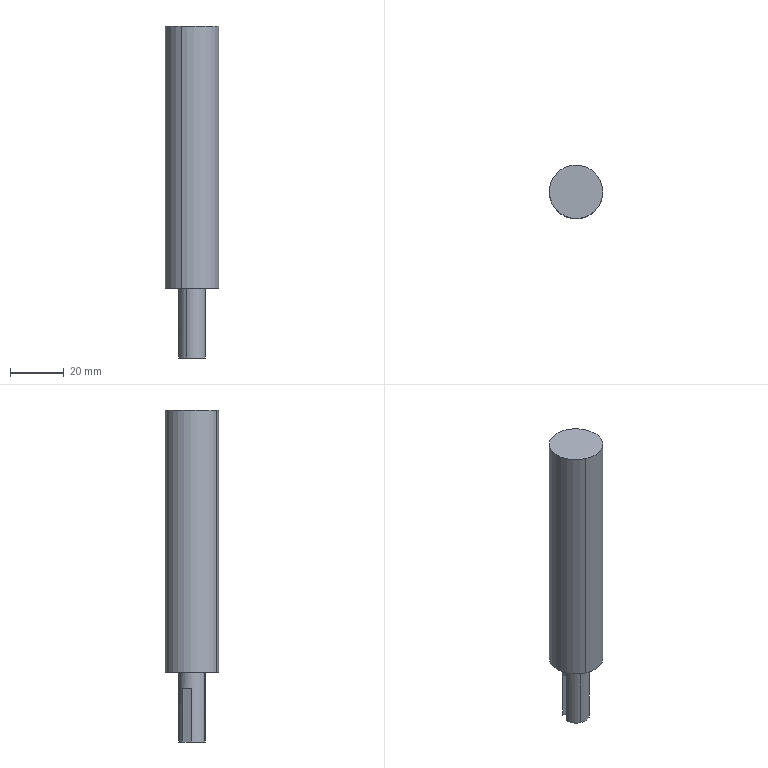Component | SolidWorks | DriveShaft-1 | 1 solid | 11 faces | box 20 x 20 x 124 mm | volume 32681 mm3 | plane 7 | cylinder 4 | commonest cylinder face diameters 10 x2 20 x2
build123d program:
from build123d import *

# Parameters (mm, degrees)
SKETCH1_R           = 10
BOSS_EXTRUDE1_DEPTH = 98
SKETCH2_R           = 5
BOSS_EXTRUDE2_DEPTH = 26
CUT_EXTRUDE1_START  = -20
CUT_EXTRUDE1_DEPTH  = 20


with BuildPart() as part:
    # Sketch1 → Boss-Extrude1 (new body)
    with BuildSketch(Plane.XY):
        Circle(SKETCH1_R)
    extrude(amount=BOSS_EXTRUDE1_DEPTH)

    # Sketch2 → Boss-Extrude2 (add)
    with BuildSketch(Plane(origin=(0, 0, 0), x_dir=(-1, 0, 0), z_dir=(0, 0, -1))):
        with Locations(Location((0, 0, 0), (0, 0, 180))):
            Circle(SKETCH2_R)
    extrude(amount=BOSS_EXTRUDE2_DEPTH)

    # Sketch3 → Cut-Extrude1 (cut)
    with BuildSketch(Plane(origin=(0, 0, -26), x_dir=(-1, 0, 0), z_dir=(0, 0, -1)).offset(CUT_EXTRUDE1_START)):
        with BuildLine():
            Line((-2, 4.583), (-2, 3))
            Line((-2, 3), (2, 3))
            Line((2, 3), (2, 4.583))
            ThreePointArc((2, 4.583), (0, 5), (-2, 4.583))
        make_face()
    extrude(amount=CUT_EXTRUDE1_DEPTH, mode=Mode.SUBTRACT)


solid = part.part

# Placed as in the assembly
solid = solid.moved(Location((28.961, 11.679, 142.846), (0, 0, 66.405)))
STEP:
#1=COLOUR_RGB('',0.7922,0.8196,0.9333);
#2=FILL_AREA_STYLE_COLOUR('',#1);
#3=FILL_AREA_STYLE('',(#2));
#4=SURFACE_STYLE_FILL_AREA(#3);
#5=SURFACE_SIDE_STYLE('',(#4));
#6=SURFACE_STYLE_USAGE(.BOTH.,#5);
#7=PRESENTATION_STYLE_ASSIGNMENT((#6));
#8=CARTESIAN_POINT('',(1.061,0.2794,4.6));
#9=VERTEX_POINT('',#8);
#10=CARTESIAN_POINT('',(0.9434,0.4599,4.6));
#11=VERTEX_POINT('',#10);
#12=CARTESIAN_POINT('',(1.14,0.4598,4.6));
#13=DIRECTION('',(0.,-0.,-1.));
#14=DIRECTION('',(-0.4003,-0.9164,0.));
#15=AXIS2_PLACEMENT_3D('',#12,#13,#14);
#16=CIRCLE('',#15,0.1969);
#17=EDGE_CURVE('',#9,#11,#16,.T.);
#18=ORIENTED_EDGE('',*,*,#17,.F.);
#19=CARTESIAN_POINT('',(1.061,0.2794,5.624));
#20=VERTEX_POINT('',#19);
#21=CARTESIAN_POINT('',(1.061,0.2794,4.6));
#22=DIRECTION('',(-0.,0.,1.));
#23=VECTOR('',#22,39.37);
#24=LINE('',#21,#23);
#25=EDGE_CURVE('',#9,#20,#24,.T.);
#26=ORIENTED_EDGE('',*,*,#25,.T.);
#27=CARTESIAN_POINT('',(1.219,0.6402,5.624));
#28=VERTEX_POINT('',#27);
#29=CARTESIAN_POINT('',(1.14,0.4598,5.624));
#30=DIRECTION('',(0.,-0.,-1.));
#31=DIRECTION('',(-0.4003,-0.9164,0.));
#32=AXIS2_PLACEMENT_3D('',#29,#30,#31);
#33=CIRCLE('',#32,0.1969);
#34=EDGE_CURVE('',#20,#28,#33,.T.);
#35=ORIENTED_EDGE('',*,*,#34,.T.);
#36=CARTESIAN_POINT('',(1.219,0.6402,4.6));
#37=VERTEX_POINT('',#36);
#38=CARTESIAN_POINT('',(1.219,0.6402,4.6));
#39=DIRECTION('',(-0.,0.,1.));
#40=VECTOR('',#39,39.37);
#41=LINE('',#38,#40);
#42=EDGE_CURVE('',#37,#28,#41,.T.);
#43=ORIENTED_EDGE('',*,*,#42,.F.);
#44=CARTESIAN_POINT('',(1.006,0.6042,4.6));
#45=VERTEX_POINT('',#44);
#46=CARTESIAN_POINT('',(1.14,0.4598,4.6));
#47=DIRECTION('',(0.,-0.,-1.));
#48=DIRECTION('',(-0.4003,-0.9164,0.));
#49=AXIS2_PLACEMENT_3D('',#46,#47,#48);
#50=CIRCLE('',#49,0.1969);
#51=EDGE_CURVE('',#45,#37,#50,.T.);
#52=ORIENTED_EDGE('',*,*,#51,.F.);
#53=CARTESIAN_POINT('',(1.006,0.6042,5.388));
#54=VERTEX_POINT('',#53);
#55=CARTESIAN_POINT('',(1.006,0.6042,5.388));
#56=DIRECTION('',(0.,-0.,-1.));
#57=VECTOR('',#56,39.37);
#58=LINE('',#55,#57);
#59=EDGE_CURVE('',#54,#45,#58,.T.);
#60=ORIENTED_EDGE('',*,*,#59,.F.);
#61=CARTESIAN_POINT('',(0.9434,0.4599,5.388));
#62=VERTEX_POINT('',#61);
#63=CARTESIAN_POINT('',(1.14,0.4598,5.388));
#64=DIRECTION('',(0.,-0.,-1.));
#65=DIRECTION('',(-0.4003,-0.9164,0.));
#66=AXIS2_PLACEMENT_3D('',#63,#64,#65);
#67=CIRCLE('',#66,0.1969);
#68=EDGE_CURVE('',#62,#54,#67,.T.);
#69=ORIENTED_EDGE('',*,*,#68,.F.);
#70=CARTESIAN_POINT('',(0.9434,0.4599,5.388));
#71=DIRECTION('',(0.,-0.,-1.));
#72=VECTOR('',#71,39.37);
#73=LINE('',#70,#72);
#74=EDGE_CURVE('',#62,#11,#73,.T.);
#75=ORIENTED_EDGE('',*,*,#74,.T.);
#76=EDGE_LOOP('',(#18,#26,#35,#43,#52,#60,#69,#75));
#77=FACE_OUTER_BOUND('',#76,.T.);
#78=CARTESIAN_POINT('',(1.14,0.4598,4.6));
#79=DIRECTION('',(-0.,0.,1.));
#80=DIRECTION('',(0.4003,0.9164,0.));
#81=AXIS2_PLACEMENT_3D('',#78,#79,#80);
#82=CYLINDRICAL_SURFACE('',#81,0.1969);
#83=ADVANCED_FACE('',(#77),#82,.T.);
#84=CARTESIAN_POINT('',(1.298,0.8206,9.482));
#85=VERTEX_POINT('',#84);
#86=CARTESIAN_POINT('',(0.9826,0.09902,9.482));
#87=VERTEX_POINT('',#86);
#88=CARTESIAN_POINT('',(1.14,0.4598,9.482));
#89=DIRECTION('',(-0.,0.,1.));
#90=DIRECTION('',(0.4003,0.9164,0.));
#91=AXIS2_PLACEMENT_3D('',#88,#89,#90);
#92=CIRCLE('',#91,0.3937);
#93=EDGE_CURVE('',#85,#87,#92,.T.);
#94=ORIENTED_EDGE('',*,*,#93,.F.);
#95=CARTESIAN_POINT('',(1.298,0.8206,5.624));
#96=VERTEX_POINT('',#95);
#97=CARTESIAN_POINT('',(1.298,0.8206,9.482));
#98=DIRECTION('',(0.,-0.,-1.));
#99=VECTOR('',#98,39.37);
#100=LINE('',#97,#99);
#101=EDGE_CURVE('',#85,#96,#100,.T.);
#102=ORIENTED_EDGE('',*,*,#101,.T.);
#103=CARTESIAN_POINT('',(0.9826,0.09902,5.624));
#104=VERTEX_POINT('',#103);
#105=CARTESIAN_POINT('',(1.14,0.4598,5.624));
#106=DIRECTION('',(-0.,0.,1.));
#107=DIRECTION('',(0.4003,0.9164,0.));
#108=AXIS2_PLACEMENT_3D('',#105,#106,#107);
#109=CIRCLE('',#108,0.3937);
#110=EDGE_CURVE('',#96,#104,#109,.T.);
#111=ORIENTED_EDGE('',*,*,#110,.T.);
#112=CARTESIAN_POINT('',(0.9826,0.09902,9.482));
#113=DIRECTION('',(0.,-0.,-1.));
#114=VECTOR('',#113,39.37);
#115=LINE('',#112,#114);
#116=EDGE_CURVE('',#87,#104,#115,.T.);
#117=ORIENTED_EDGE('',*,*,#116,.F.);
#118=EDGE_LOOP('',(#94,#102,#111,#117));
#119=FACE_OUTER_BOUND('',#118,.T.);
#120=CARTESIAN_POINT('',(1.14,0.4598,9.482));
#121=DIRECTION('',(0.,-0.,-1.));
#122=DIRECTION('',(-0.4003,-0.9164,0.));
#123=AXIS2_PLACEMENT_3D('',#120,#121,#122);
#124=CYLINDRICAL_SURFACE('',#123,0.3937);
#125=ADVANCED_FACE('',(#119),#124,.T.);
#126=ORIENTED_EDGE('',*,*,#101,.F.);
#127=CARTESIAN_POINT('',(1.14,0.4598,9.482));
#128=DIRECTION('',(-0.,0.,1.));
#129=DIRECTION('',(0.4003,0.9164,0.));
#130=AXIS2_PLACEMENT_3D('',#127,#128,#129);
#131=CIRCLE('',#130,0.3937);
#132=EDGE_CURVE('',#87,#85,#131,.T.);
#133=ORIENTED_EDGE('',*,*,#132,.F.);
#134=ORIENTED_EDGE('',*,*,#116,.T.);
#135=CARTESIAN_POINT('',(1.14,0.4598,5.624));
#136=DIRECTION('',(-0.,0.,1.));
#137=DIRECTION('',(0.4003,0.9164,0.));
#138=AXIS2_PLACEMENT_3D('',#135,#136,#137);
#139=CIRCLE('',#138,0.3937);
#140=EDGE_CURVE('',#104,#96,#139,.T.);
#141=ORIENTED_EDGE('',*,*,#140,.T.);
#142=EDGE_LOOP('',(#126,#133,#134,#141));
#143=FACE_OUTER_BOUND('',#142,.T.);
#144=CARTESIAN_POINT('',(1.14,0.4598,9.482));
#145=DIRECTION('',(0.,-0.,-1.));
#146=DIRECTION('',(-0.4003,-0.9164,0.));
#147=AXIS2_PLACEMENT_3D('',#144,#145,#146);
#148=CYLINDRICAL_SURFACE('',#147,0.3937);
#149=ADVANCED_FACE('',(#143),#148,.T.);
#150=ORIENTED_EDGE('',*,*,#132,.T.);
#151=ORIENTED_EDGE('',*,*,#93,.T.);
#152=EDGE_LOOP('',(#150,#151));
#153=FACE_OUTER_BOUND('',#152,.T.);
#154=CARTESIAN_POINT('',(1.14,0.4598,9.482));
#155=DIRECTION('',(-0.,0.,1.));
#156=DIRECTION('',(0.4003,0.9164,0.));
#157=AXIS2_PLACEMENT_3D('',#154,#155,#156);
#158=PLANE('',#157);
#159=ADVANCED_FACE('',(#153),#158,.T.);
#160=CARTESIAN_POINT('',(1.14,0.4598,5.624));
#161=DIRECTION('',(0.,-0.,-1.));
#162=DIRECTION('',(-0.4003,-0.9164,0.));
#163=AXIS2_PLACEMENT_3D('',#160,#161,#162);
#164=CIRCLE('',#163,0.1969);
#165=EDGE_CURVE('',#28,#20,#164,.T.);
#166=ORIENTED_EDGE('',*,*,#165,.F.);
#167=ORIENTED_EDGE('',*,*,#34,.F.);
#168=EDGE_LOOP('',(#166,#167));
#169=FACE_BOUND('',#168,.T.);
#170=ORIENTED_EDGE('',*,*,#140,.F.);
#171=ORIENTED_EDGE('',*,*,#110,.F.);
#172=EDGE_LOOP('',(#170,#171));
#173=FACE_OUTER_BOUND('',#172,.T.);
#174=CARTESIAN_POINT('',(1.14,0.4598,5.624));
#175=DIRECTION('',(-0.,0.,1.));
#176=DIRECTION('',(0.4003,0.9164,0.));
#177=AXIS2_PLACEMENT_3D('',#174,#175,#176);
#178=PLANE('',#177);
#179=ADVANCED_FACE('',(#169,#173),#178,.F.);
#180=ORIENTED_EDGE('',*,*,#25,.F.);
#181=CARTESIAN_POINT('',(1.14,0.4598,4.6));
#182=DIRECTION('',(0.,-0.,-1.));
#183=DIRECTION('',(-0.4003,-0.9164,0.));
#184=AXIS2_PLACEMENT_3D('',#181,#182,#183);
#185=CIRCLE('',#184,0.1969);
#186=EDGE_CURVE('',#37,#9,#185,.T.);
#187=ORIENTED_EDGE('',*,*,#186,.F.);
#188=ORIENTED_EDGE('',*,*,#42,.T.);
#189=ORIENTED_EDGE('',*,*,#165,.T.);
#190=EDGE_LOOP('',(#180,#187,#188,#189));
#191=FACE_OUTER_BOUND('',#190,.T.);
#192=CARTESIAN_POINT('',(1.14,0.4598,4.6));
#193=DIRECTION('',(-0.,0.,1.));
#194=DIRECTION('',(0.4003,0.9164,0.));
#195=AXIS2_PLACEMENT_3D('',#192,#193,#194);
#196=CYLINDRICAL_SURFACE('',#195,0.1969);
#197=ADVANCED_FACE('',(#191),#196,.T.);
#198=CARTESIAN_POINT('',(1.063,0.5792,4.6));
#199=VERTEX_POINT('',#198);
#200=CARTESIAN_POINT('',(1.006,0.6042,4.6));
#201=DIRECTION('',(0.9164,-0.4003,0.));
#202=VECTOR('',#201,39.37);
#203=LINE('',#200,#202);
#204=EDGE_CURVE('',#45,#199,#203,.T.);
#205=ORIENTED_EDGE('',*,*,#204,.F.);
#206=ORIENTED_EDGE('',*,*,#51,.T.);
#207=ORIENTED_EDGE('',*,*,#186,.T.);
#208=ORIENTED_EDGE('',*,*,#17,.T.);
#209=CARTESIAN_POINT('',(1.,0.4349,4.6));
#210=VERTEX_POINT('',#209);
#211=CARTESIAN_POINT('',(0.9434,0.4599,4.6));
#212=DIRECTION('',(-0.9164,0.4003,-0.));
#213=VECTOR('',#212,39.37);
#214=LINE('',#211,#213);
#215=EDGE_CURVE('',#210,#11,#214,.T.);
#216=ORIENTED_EDGE('',*,*,#215,.F.);
#217=CARTESIAN_POINT('',(1.,0.4349,4.6));
#218=DIRECTION('',(-0.4003,-0.9164,-0.));
#219=VECTOR('',#218,39.37);
#220=LINE('',#217,#219);
#221=EDGE_CURVE('',#199,#210,#220,.T.);
#222=ORIENTED_EDGE('',*,*,#221,.F.);
#223=EDGE_LOOP('',(#205,#206,#207,#208,#216,#222));
#224=FACE_OUTER_BOUND('',#223,.T.);
#225=CARTESIAN_POINT('',(1.14,0.4598,4.6));
#226=DIRECTION('',(0.,-0.,-1.));
#227=DIRECTION('',(-0.4003,-0.9164,-0.));
#228=AXIS2_PLACEMENT_3D('',#225,#226,#227);
#229=PLANE('',#228);
#230=ADVANCED_FACE('',(#224),#229,.T.);
#231=ORIENTED_EDGE('',*,*,#221,.T.);
#232=CARTESIAN_POINT('',(1.,0.4349,5.388));
#233=VERTEX_POINT('',#232);
#234=CARTESIAN_POINT('',(1.,0.4349,5.388));
#235=DIRECTION('',(0.,-0.,-1.));
#236=VECTOR('',#235,39.37);
#237=LINE('',#234,#236);
#238=EDGE_CURVE('',#233,#210,#237,.T.);
#239=ORIENTED_EDGE('',*,*,#238,.F.);
#240=CARTESIAN_POINT('',(1.063,0.5792,5.388));
#241=VERTEX_POINT('',#240);
#242=CARTESIAN_POINT('',(1.,0.4349,5.388));
#243=DIRECTION('',(-0.4003,-0.9164,-0.));
#244=VECTOR('',#243,39.37);
#245=LINE('',#242,#244);
#246=EDGE_CURVE('',#241,#233,#245,.T.);
#247=ORIENTED_EDGE('',*,*,#246,.F.);
#248=CARTESIAN_POINT('',(1.063,0.5792,5.388));
#249=DIRECTION('',(0.,-0.,-1.));
#250=VECTOR('',#249,39.37);
#251=LINE('',#248,#250);
#252=EDGE_CURVE('',#241,#199,#251,.T.);
#253=ORIENTED_EDGE('',*,*,#252,.T.);
#254=EDGE_LOOP('',(#231,#239,#247,#253));
#255=FACE_OUTER_BOUND('',#254,.T.);
#256=CARTESIAN_POINT('',(1.,0.4349,5.388));
#257=DIRECTION('',(0.9164,-0.4003,0.));
#258=DIRECTION('',(0.4003,0.9164,0.));
#259=AXIS2_PLACEMENT_3D('',#256,#257,#258);
#260=PLANE('',#259);
#261=ADVANCED_FACE('',(#255),#260,.F.);
#262=ORIENTED_EDGE('',*,*,#204,.T.);
#263=ORIENTED_EDGE('',*,*,#252,.F.);
#264=CARTESIAN_POINT('',(1.006,0.6042,5.388));
#265=DIRECTION('',(0.9164,-0.4003,0.));
#266=VECTOR('',#265,39.37);
#267=LINE('',#264,#266);
#268=EDGE_CURVE('',#54,#241,#267,.T.);
#269=ORIENTED_EDGE('',*,*,#268,.F.);
#270=ORIENTED_EDGE('',*,*,#59,.T.);
#271=EDGE_LOOP('',(#262,#263,#269,#270));
#272=FACE_OUTER_BOUND('',#271,.T.);
#273=CARTESIAN_POINT('',(1.006,0.6042,5.388));
#274=DIRECTION('',(0.4003,0.9164,0.));
#275=DIRECTION('',(-0.9164,0.4003,-0.));
#276=AXIS2_PLACEMENT_3D('',#273,#274,#275);
#277=PLANE('',#276);
#278=ADVANCED_FACE('',(#272),#277,.F.);
#279=ORIENTED_EDGE('',*,*,#215,.T.);
#280=ORIENTED_EDGE('',*,*,#74,.F.);
#281=CARTESIAN_POINT('',(0.9434,0.4599,5.388));
#282=DIRECTION('',(-0.9164,0.4003,-0.));
#283=VECTOR('',#282,39.37);
#284=LINE('',#281,#283);
#285=EDGE_CURVE('',#233,#62,#284,.T.);
#286=ORIENTED_EDGE('',*,*,#285,.F.);
#287=ORIENTED_EDGE('',*,*,#238,.T.);
#288=EDGE_LOOP('',(#279,#280,#286,#287));
#289=FACE_OUTER_BOUND('',#288,.T.);
#290=CARTESIAN_POINT('',(0.9434,0.4599,5.388));
#291=DIRECTION('',(-0.4003,-0.9164,-0.));
#292=DIRECTION('',(-0.,0.,1.));
#293=AXIS2_PLACEMENT_3D('',#290,#291,#292);
#294=PLANE('',#293);
#295=ADVANCED_FACE('',(#289),#294,.F.);
#296=ORIENTED_EDGE('',*,*,#246,.T.);
#297=ORIENTED_EDGE('',*,*,#285,.T.);
#298=ORIENTED_EDGE('',*,*,#68,.T.);
#299=ORIENTED_EDGE('',*,*,#268,.T.);
#300=EDGE_LOOP('',(#296,#297,#298,#299));
#301=FACE_OUTER_BOUND('',#300,.T.);
#302=CARTESIAN_POINT('',(1.14,0.4598,5.388));
#303=DIRECTION('',(0.,-0.,-1.));
#304=DIRECTION('',(-0.4003,-0.9164,-0.));
#305=AXIS2_PLACEMENT_3D('',#302,#303,#304);
#306=PLANE('',#305);
#307=ADVANCED_FACE('',(#301),#306,.T.);
#308=CLOSED_SHELL('',(#83,#125,#149,#159,#179,#197,#230,#261,#278,#295,#307));
#309=MANIFOLD_SOLID_BREP('',#308);
#310=STYLED_ITEM('',(#7),#309);
#311=(LENGTH_UNIT()NAMED_UNIT(*)SI_UNIT($,.METRE.));
#312=LENGTH_MEASURE_WITH_UNIT(LENGTH_MEASURE(0.0254),#311);
#313=DIMENSIONAL_EXPONENTS(1.,0.,0.,0.,0.,0.,0.);
#314=(CONVERSION_BASED_UNIT('',#312)LENGTH_UNIT()NAMED_UNIT(#313));
#315=UNCERTAINTY_MEASURE_WITH_UNIT(LENGTH_MEASURE(0.00001),#314,'','');
#316=(NAMED_UNIT(*)PLANE_ANGLE_UNIT()SI_UNIT($,.RADIAN.));
#317=(NAMED_UNIT(*)SI_UNIT($,.STERADIAN.)SOLID_ANGLE_UNIT());
#318=(GEOMETRIC_REPRESENTATION_CONTEXT(3)GLOBAL_UNCERTAINTY_ASSIGNED_CONTEXT((#315))GLOBAL_UNIT_ASSIGNED_CONTEXT((#314,#316,#317))REPRESENTATION_CONTEXT('',''));
#319=MECHANICAL_DESIGN_GEOMETRIC_PRESENTATION_REPRESENTATION('',(#310),#318);
#320=CARTESIAN_POINT('',(0.,0.,0.));
#321=DIRECTION('',(0.,0.,1.));
#322=DIRECTION('',(1.,0.,0.));
#323=AXIS2_PLACEMENT_3D('',#320,#321,#322);
#324=(LENGTH_UNIT()NAMED_UNIT(*)SI_UNIT($,.METRE.));
#325=LENGTH_MEASURE_WITH_UNIT(LENGTH_MEASURE(0.0254),#324);
#326=DIMENSIONAL_EXPONENTS(1.,0.,0.,0.,0.,0.,0.);
#327=(CONVERSION_BASED_UNIT('',#325)LENGTH_UNIT()NAMED_UNIT(#326));
#328=UNCERTAINTY_MEASURE_WITH_UNIT(LENGTH_MEASURE(0.00001),#327,'','');
#329=(NAMED_UNIT(*)PLANE_ANGLE_UNIT()SI_UNIT($,.RADIAN.));
#330=(NAMED_UNIT(*)SI_UNIT($,.STERADIAN.)SOLID_ANGLE_UNIT());
#331=(GEOMETRIC_REPRESENTATION_CONTEXT(3)GLOBAL_UNCERTAINTY_ASSIGNED_CONTEXT((#328))GLOBAL_UNIT_ASSIGNED_CONTEXT((#327,#329,#330))REPRESENTATION_CONTEXT('',''));
#332=ADVANCED_BREP_SHAPE_REPRESENTATION('',(#309,#323),#331);
#333=PRESENTATION_LAYER_ASSIGNMENT('','',(#310));